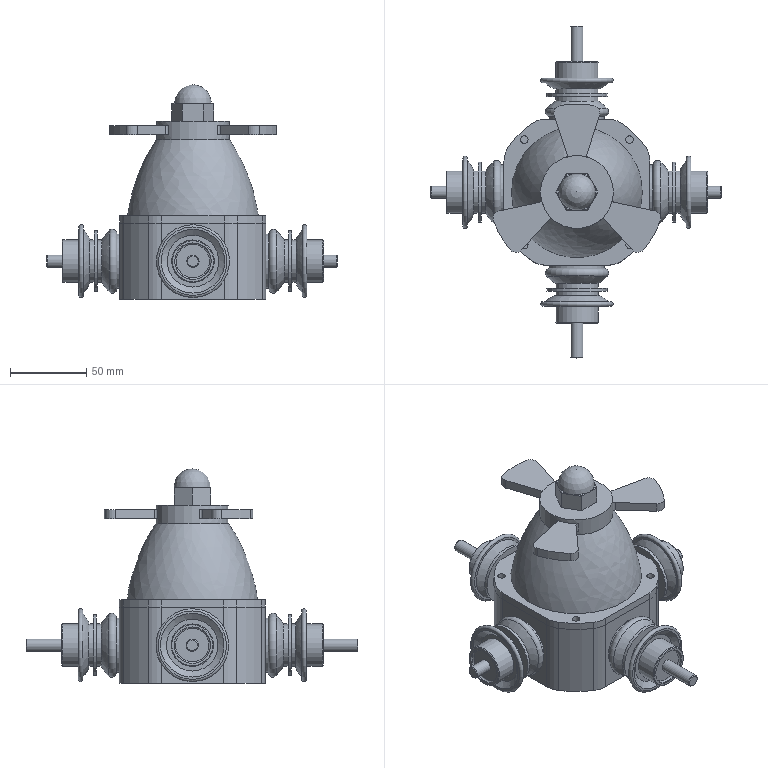Assembly | NX | mm | 27 component files | 46 solids | 715 faces | box 191.12 x 218.36 x 141 mm | volume 455332 mm3 | plane 312 | cylinder 260 | cone 75 | spline 27 | torus 22 | sphere 19 | commonest cylinder face diameters 32 x24 5 x24 24 x24 0.4 x24 20 x19 8 x17 28 x13 12 x11
Bill of materials:
unnamed part 1 | 4 |  | Short thick-walled cylindrical ring (annular sleeve) with a plain through bore and chamfered outer edges at both end faces.
unnamed part 2 | 4 |  | Hollow revolved sleeve with a central cylindrical body, plain tubular ends of slightly different diameters, a rounded bulbous collar, a thin flat disk-like ring, and a flared conical lip with rounded rim.
unnamed part 3 | 1 |  | Dome/bell-shaped hollow-looking shell with flat-topped truncated crown and central through hole, rising from a thin flat base flange with chamfered square-octagonal outline and four small holes near the corners.
unnamed part 4 | 4 |  | Cylindrical tube/sleeve, roughly as long as its diameter, with a through bore and chamfers on outer edges and bore edges.
unnamed part 5 | 4 |  | Hex-head bolt-like part: hexagonal head with a plain cylindrical shank ending in a chamfered tip.
unnamed part 6 | 1 |  | Flat three-lobed plate with a thicker central annular hub and round through hole; three tapered, rounded-tip arms radiate at roughly equal angular spacing.
unnamed part 7 | 1 |  | Complex revolved body with through bore: external thread-like ridges at the top end, stepped tapering cylindrical sections, multiple thin flanges, a conical flare, a rounded bulge, a set of thin closely spaced fins/rings, a lower cylindrical section with rectangular notches, and a two-lobed flat base flange.
unnamed part 8 | 4 |  | Clevis-ended cylindrical body with a protruding rod: a two-tine fork with cross holes at one end, a stepped cylindrical housing with several circumferential grooves, and a long plain round rod extending from the opposite face.
unnamed part 9 | 1 |  | Ball-bearing-like ring assembly: outer ring and inner ring separated by an annular gap containing a ring of spherical elements, with chamfered outer edges.
unnamed part 10 | 1 |  | Acorn/cap-nut-like part: hexagonal prism base with a hemispherical dome on top.
unnamed part 11 | 1 |  | Solid stepped revolved pin with a thin radial flange: small top cylinder, larger middle cylinder, flange disc, and a lower cylinder, all with chamfered edges.
unnamed part 12 | 1 |  | Open-top box-like housing with rounded-square/clipped-corner outline, a thin top rim with four small holes, a large round port with protruding boss on each of four sides, and a floor with three curved arc slots around a small center hole.
Mates:
1. fix | base 1 component
2. concentric | support_shaft 1 edge | base 1 arc
3. concentric | roller 4 arc | piston 4 edge
4. touch align | piston 4 face | base 1 face
5. parallel | piston 4 face | camshaft 1 face
6. touch align | camshaft 1 face | support_shaft 1 face
7. center | camshaft 1 face | camshaft 1 face | piston 4 face | piston 4 face
8. concentric | roller 3 arc | piston 3 edge
9. touch align | piston 3 face | base 1 face
10. parallel | piston 3 face | camshaft 1 face
11. concentric | roller 2 arc | piston 2 edge
12. touch align | piston 2 face | base 1 face
13. parallel | piston 2 face | camshaft 1 face
14. concentric | roller 1 arc | piston 1 edge
15. touch align | piston 1 face | base 1 face
16. parallel | piston 1 face | piston 2 face
17. concentric | cylinder_block 4 edge | base 1 edge
18. fix | assembly component
19. bond | cylinder_block 4 component | assembly component
20. bond | cylinder_block 3 component | assembly component
21. bond | cylinder_block 2 component | assembly component
22. bond | cylinder_block 1 component | assembly component
23. circular | assembly datumaxis | assembly cartesiancoordinatesystem | assembly cartesiancoordinatesystem | assembly cartesiancoordinatesystem | assembly cartesiancoordinatesystem
24. concentric | base 1 arc | top_cover 1 arc
25. parallel | base 1 face | top_cover 1 face
26. concentric | impeller 1 edge | top_cover 1 arc
27. concentric | impeller 1 edge | nut_cap 1 arc
28. parallel | nut_cap 1 face | top_cover 1 face
29. concentric | camshaft 1 edge | bearing 1 edge
30. concentric | bolt 4 edge | piston 1 edge
31. concentric | piston 3 edge | bolt 3 edge
32. concentric | piston 2 edge | bolt 2 edge
33. concentric | piston 4 edge | bolt 1 edge
34. concentric | nut 4 arc | piston 1 edge
35. concentric | nut 3 arc | piston 4 edge
36. concentric | nut 2 arc | piston 3 edge
37. concentric | nut 1 arc | piston 2 edge